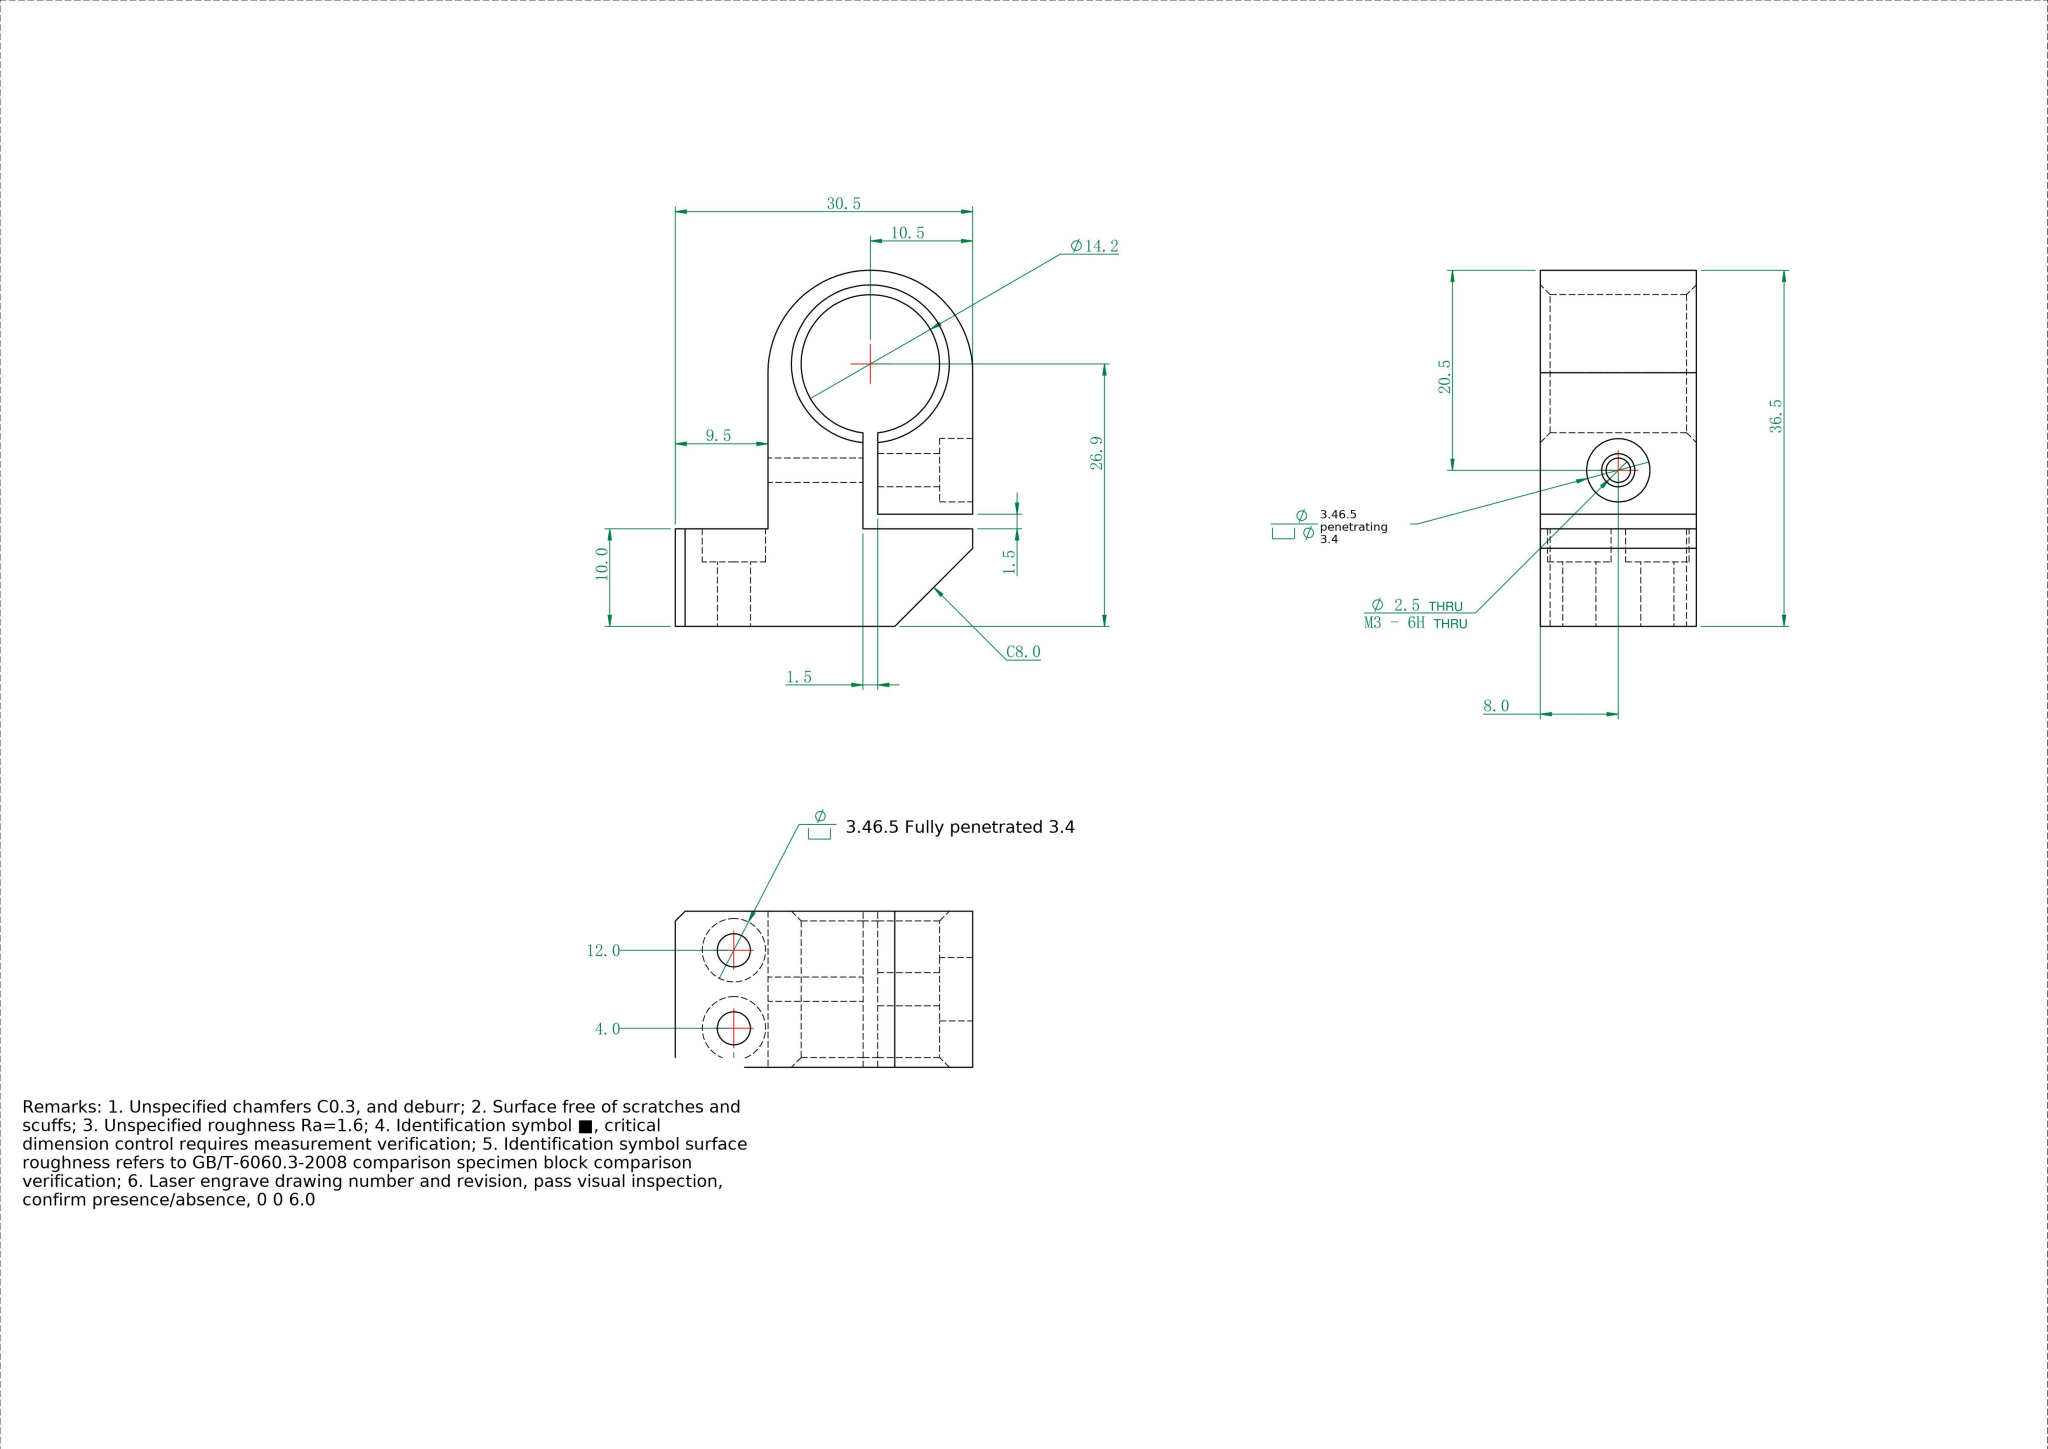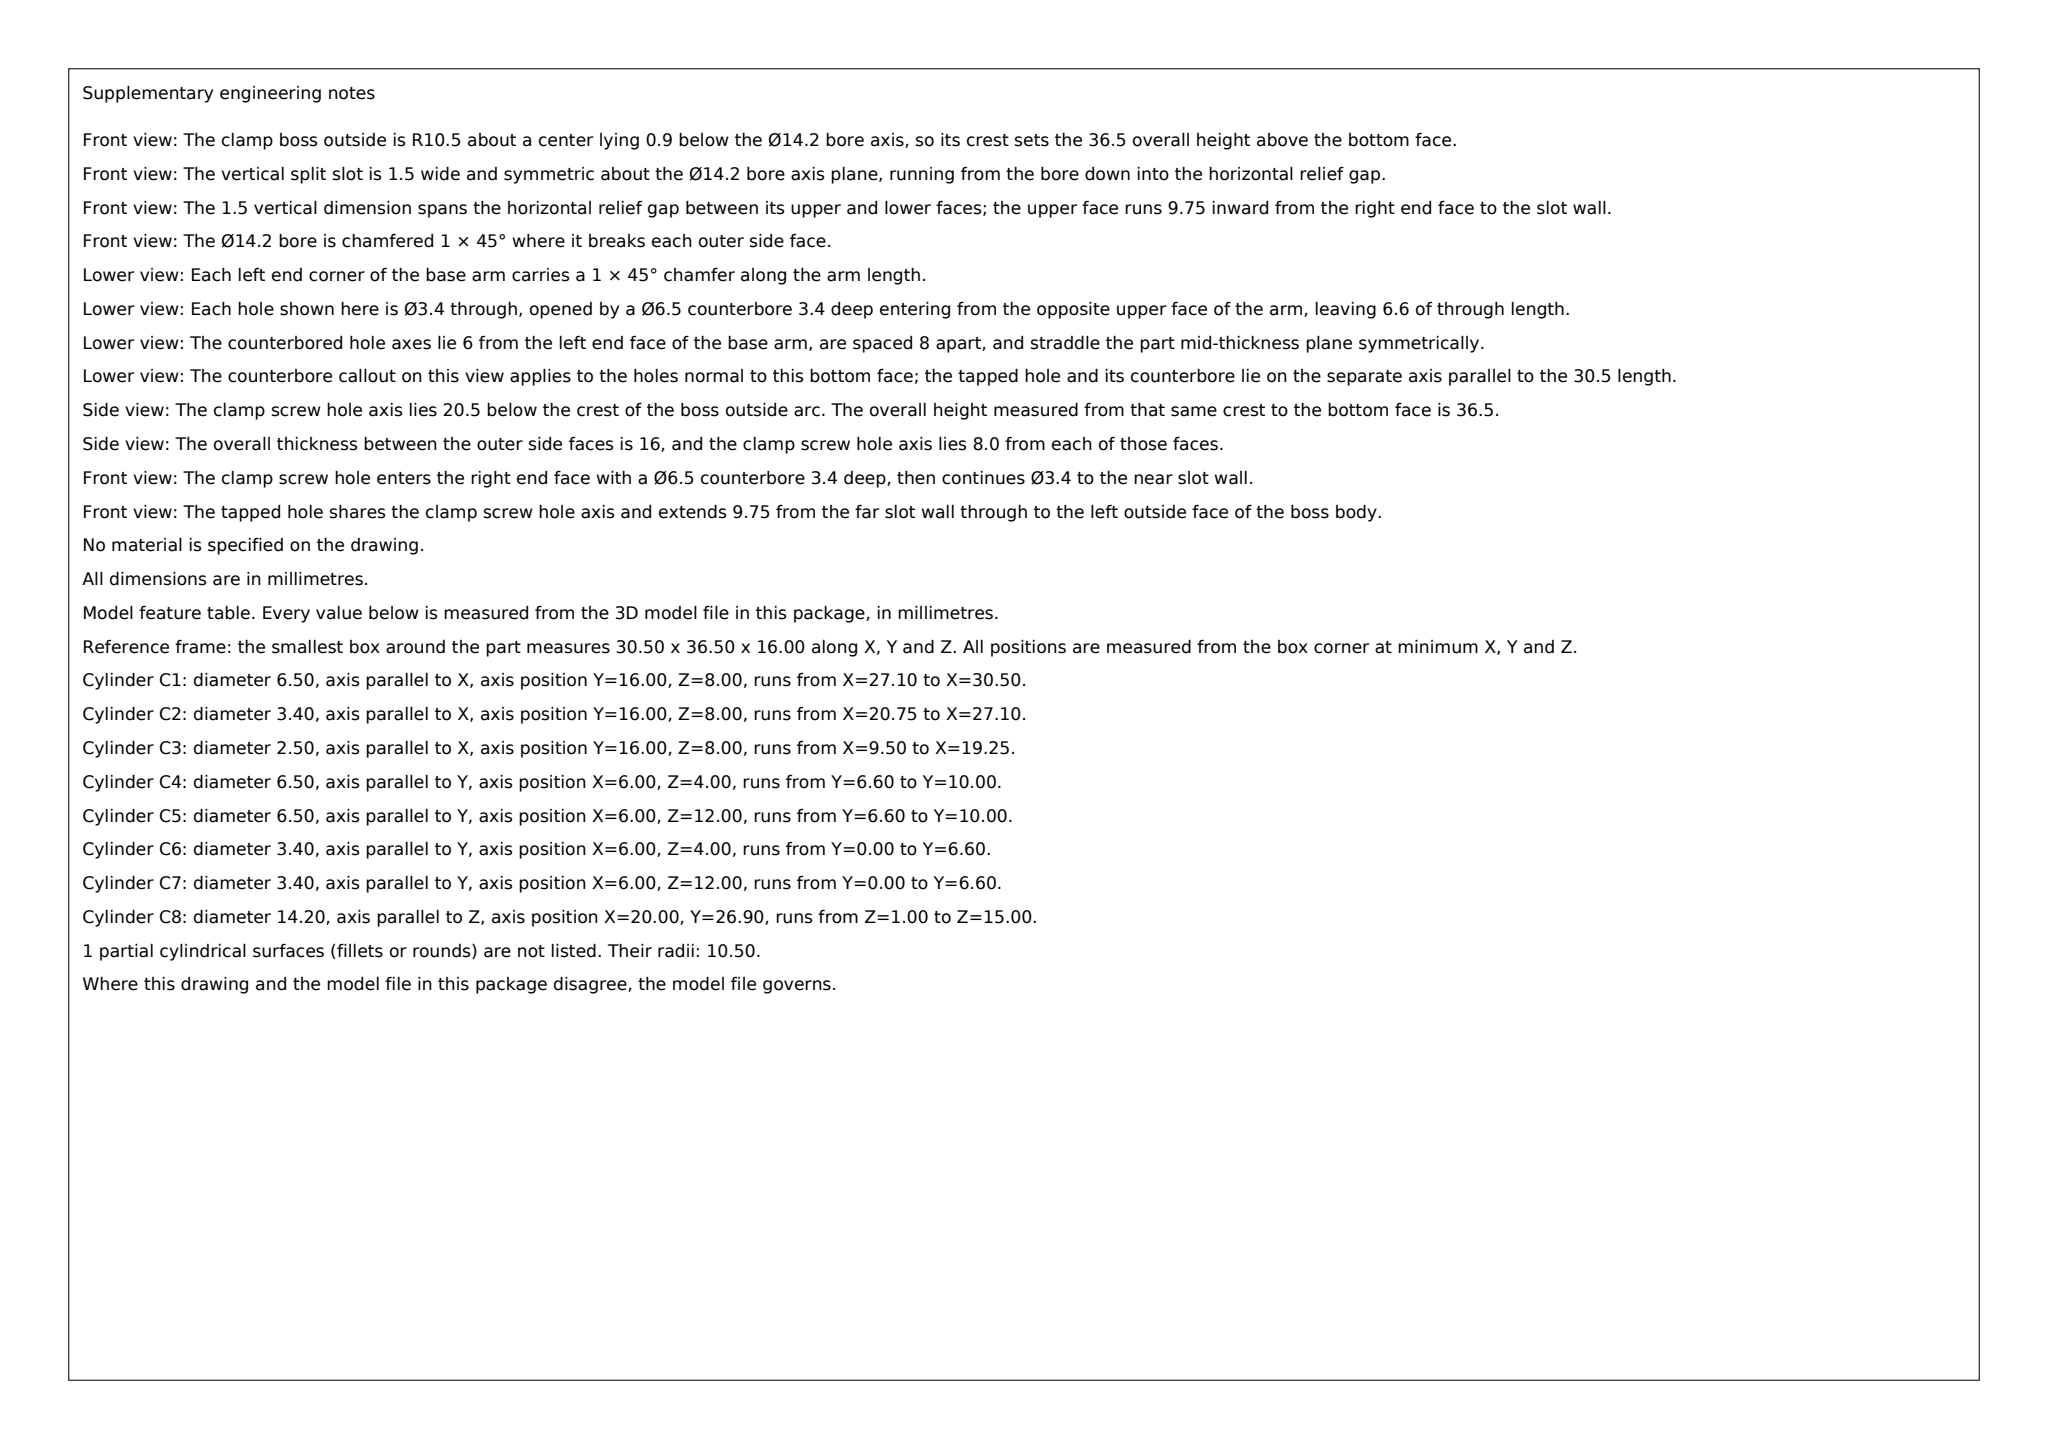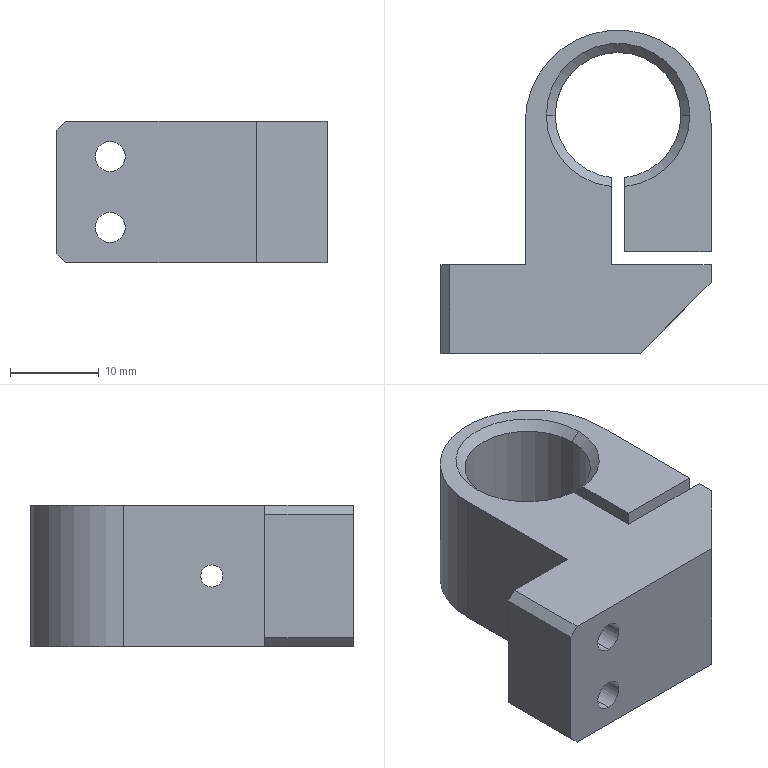Part | SolidWorks | mm | 1 solid | 42 faces | box 30.5 x 36.5 x 16 mm | volume 8892 mm3 | cylinder 18 | plane 18 | cone 6 | commonest cylinder face diameters 6.5 x6 3.4 x6 14.2 x3 2.5 x2 21 x1
Drawing notes:
STOCK 30.5 X 36.5 X 16.0 | from the solid: bbox_xyz [30.5,36.5,16.0]
STEP 1.5 HIGH ABV 10.0 BASE (TOP 11.5), X9.5 TO X27.1 | from the solid: y planes 10.0 & 11.5; x planes 9.5 & 27.1
CLAMP HEAD OD Ø21.0, ARC CL 26.0 ABV BASE (0.9 BELOW Ø14.2 CL 26.9) | from the solid: cyl Ø21.0 axis z at [20.0,26.0]; Ø14.2 bore at [20.0,26.9]
CLAMP SLOT 1.5 WIDE THRU, SYM ABOUT Ø14.2 BORE CL X=20.0 | from the solid: x planes 19.25 & 20.75 = 1.5 gap centered on bore axis x=20.0
2X Ø3.4 THRU BASE, CBORE Ø6.5 DP 3.4 BOTH ENDS, AT X6.0, Z4.0 & Z12.0 | from the solid: cyl 3.4 axis y at (6.0,4.0) & (6.0,12.0) L6.6; cyl 6.5 axis y same pos L3.4, 2 ea
SIDE HOLE CL Y16.0, Z8.0: Ø2.5 THRU, M3-6H; Ø3.4 DP 9.75 EA END | from the solid: cyl 2.5 axis x (y16,z8) L9.75; cyl 3.4 axis x L6.35 behind Ø6.5 CBORE 3.4
SIDE HOLE CBORE Ø6.5 DP 3.4 BOTH ENDS; M3 THD LG 11.0 CTR OF 30.5 | from the solid: cyl 6.5 axis x L3.4 count 2; 30.5-2x9.75=11.0 central Ø2.5 section
build123d program:
from build123d import *

# Parameters (mm, degrees)
BOSS_EXTRUDE1_DEPTH                             = 16
SKETCH2_W                                       = 16
SKETCH2_H                                       = 10
BOSS_EXTRUDE2_DEPTH                             = 9.5
CUT_EXTRUDE1_DEPTH                              = 32.449
SKETCH4_W                                       = 7.1
SKETCH4_H                                       = 16
M3_HEX_SOCKET_HEAD_CAP_SCREW_CBORE1_D           = 3.4
M3_HEX_SOCKET_HEAD_CAP_SCREW_CBORE1_CBORE_D     = 6.5
M3_HEX_SOCKET_HEAD_CAP_SCREW_CBORE1_CBORE_DEPTH = 3.4
M3_TAPPED_HOLE1_D                               = 2.5
M3_TAPPED_HOLE1_DEPTH                           = 9.75
M3_HEX_SOCKET_HEAD_CAP_SCREW_CBORE2_D           = 3.4
M3_HEX_SOCKET_HEAD_CAP_SCREW_CBORE2_DEPTH       = 9.75
M3_HEX_SOCKET_HEAD_CAP_SCREW_CBORE2_CBORE_D     = 6.5
M3_HEX_SOCKET_HEAD_CAP_SCREW_CBORE2_CBORE_DEPTH = 3.4
CHAMFER1_SIZE                                   = 1
CHAMFER2_SIZE                                   = 8


with BuildPart() as part:
    # Sketch1 → Boss-Extrude1 (new body)
    with BuildSketch(Plane(origin=(0, 0, -8), x_dir=(-1, 0, 0), z_dir=(0, 0, -1))):
        with BuildLine():
            Line((-10.5, -18.25), (10.5, -18.25))
            Line((10.5, -18.25), (10.5, 7.75))
            ThreePointArc((10.5, 7.75), (0, 18.25), (-10.5, 7.75))
            Line((-10.5, 7.75), (-10.5, -18.25))
        make_face()
    extrude(amount=-BOSS_EXTRUDE1_DEPTH)

    # Sketch2 → Boss-Extrude2 (add)
    with BuildSketch(Plane.ZY.offset(10.5)):
        with Locations((0, -13.25)):
            Rectangle(SKETCH2_W, SKETCH2_H)
    extrude(amount=BOSS_EXTRUDE2_DEPTH)

    # Sketch3 → Cut-Extrude1 (cut, through all)
    with BuildSketch(Plane.XY.offset(8)):
        with BuildLine():
            Line((10.5, -8.25), (10.5, -6.75))
            Line((10.5, -6.75), (0.75, -6.75))
            Line((0.75, -6.75), (0.75, 1.59))
            ThreePointArc((0.75, 1.59), (0, 1.55), (-0.75, 1.59))
            Line((-0.75, 1.59), (-0.75, -8.25))
            Line((-0.75, -8.25), (10.5, -8.25))
        make_face()
    extrude(amount=-CUT_EXTRUDE1_DEPTH, mode=Mode.SUBTRACT)

    # Sketch4 → Cut-Revolve1 (revolve, cut)
    with BuildSketch(Plane(origin=(0, 8.65, 0), x_dir=(1, 0, 0), z_dir=(0, 1, 0))):
        with Locations((3.55, 0)):
            Rectangle(SKETCH4_W, SKETCH4_H)
    revolve(axis=Axis((0, 8.65, -8), (0, 0, 1)), mode=Mode.SUBTRACT)

    # M3 Hex Socket Head Cap Screw CBORE1 (through all)
    with Locations(Plane(origin=(0, -8.25, 0), x_dir=(1, 0, 0), z_dir=(0, 1, 0))):
        with Locations((-14, -4), (-14, 4)):
            CounterBoreHole(M3_HEX_SOCKET_HEAD_CAP_SCREW_CBORE1_D / 2, M3_HEX_SOCKET_HEAD_CAP_SCREW_CBORE1_CBORE_D / 2, M3_HEX_SOCKET_HEAD_CAP_SCREW_CBORE1_CBORE_DEPTH)

    # M3 Tapped Hole1
    with Locations(Plane.ZY.offset(10.5)):
        with Locations((0, -2.25)):
            Hole(M3_TAPPED_HOLE1_D / 2, depth=M3_TAPPED_HOLE1_DEPTH)

    # M3 Hex Socket Head Cap Screw CBORE2
    with Locations(Plane(origin=(10.5, 0, 0), x_dir=(0, 0, -1), z_dir=(1, 0, 0))):
        with Locations((0, -2.25)):
            CounterBoreHole(M3_HEX_SOCKET_HEAD_CAP_SCREW_CBORE2_D / 2, M3_HEX_SOCKET_HEAD_CAP_SCREW_CBORE2_CBORE_D / 2, M3_HEX_SOCKET_HEAD_CAP_SCREW_CBORE2_CBORE_DEPTH, depth=M3_HEX_SOCKET_HEAD_CAP_SCREW_CBORE2_DEPTH)

    # Chamfer1
    chamfer1_edges = [part.edges().sort_by_distance(p)[0] for p in [
        (-20, -13.25, -8),
        (-20, -13.25, 8),
        (0, 15.75, -8),
        (0, 15.75, 8),
    ]]
    chamfer(chamfer1_edges, length=CHAMFER1_SIZE)

    # Chamfer2
    chamfer2_edges = [part.edges().sort_by_distance(p)[0] for p in [
        (10.5, -18.25, 0),
    ]]
    chamfer(chamfer2_edges, length=CHAMFER2_SIZE)


solid = part.part